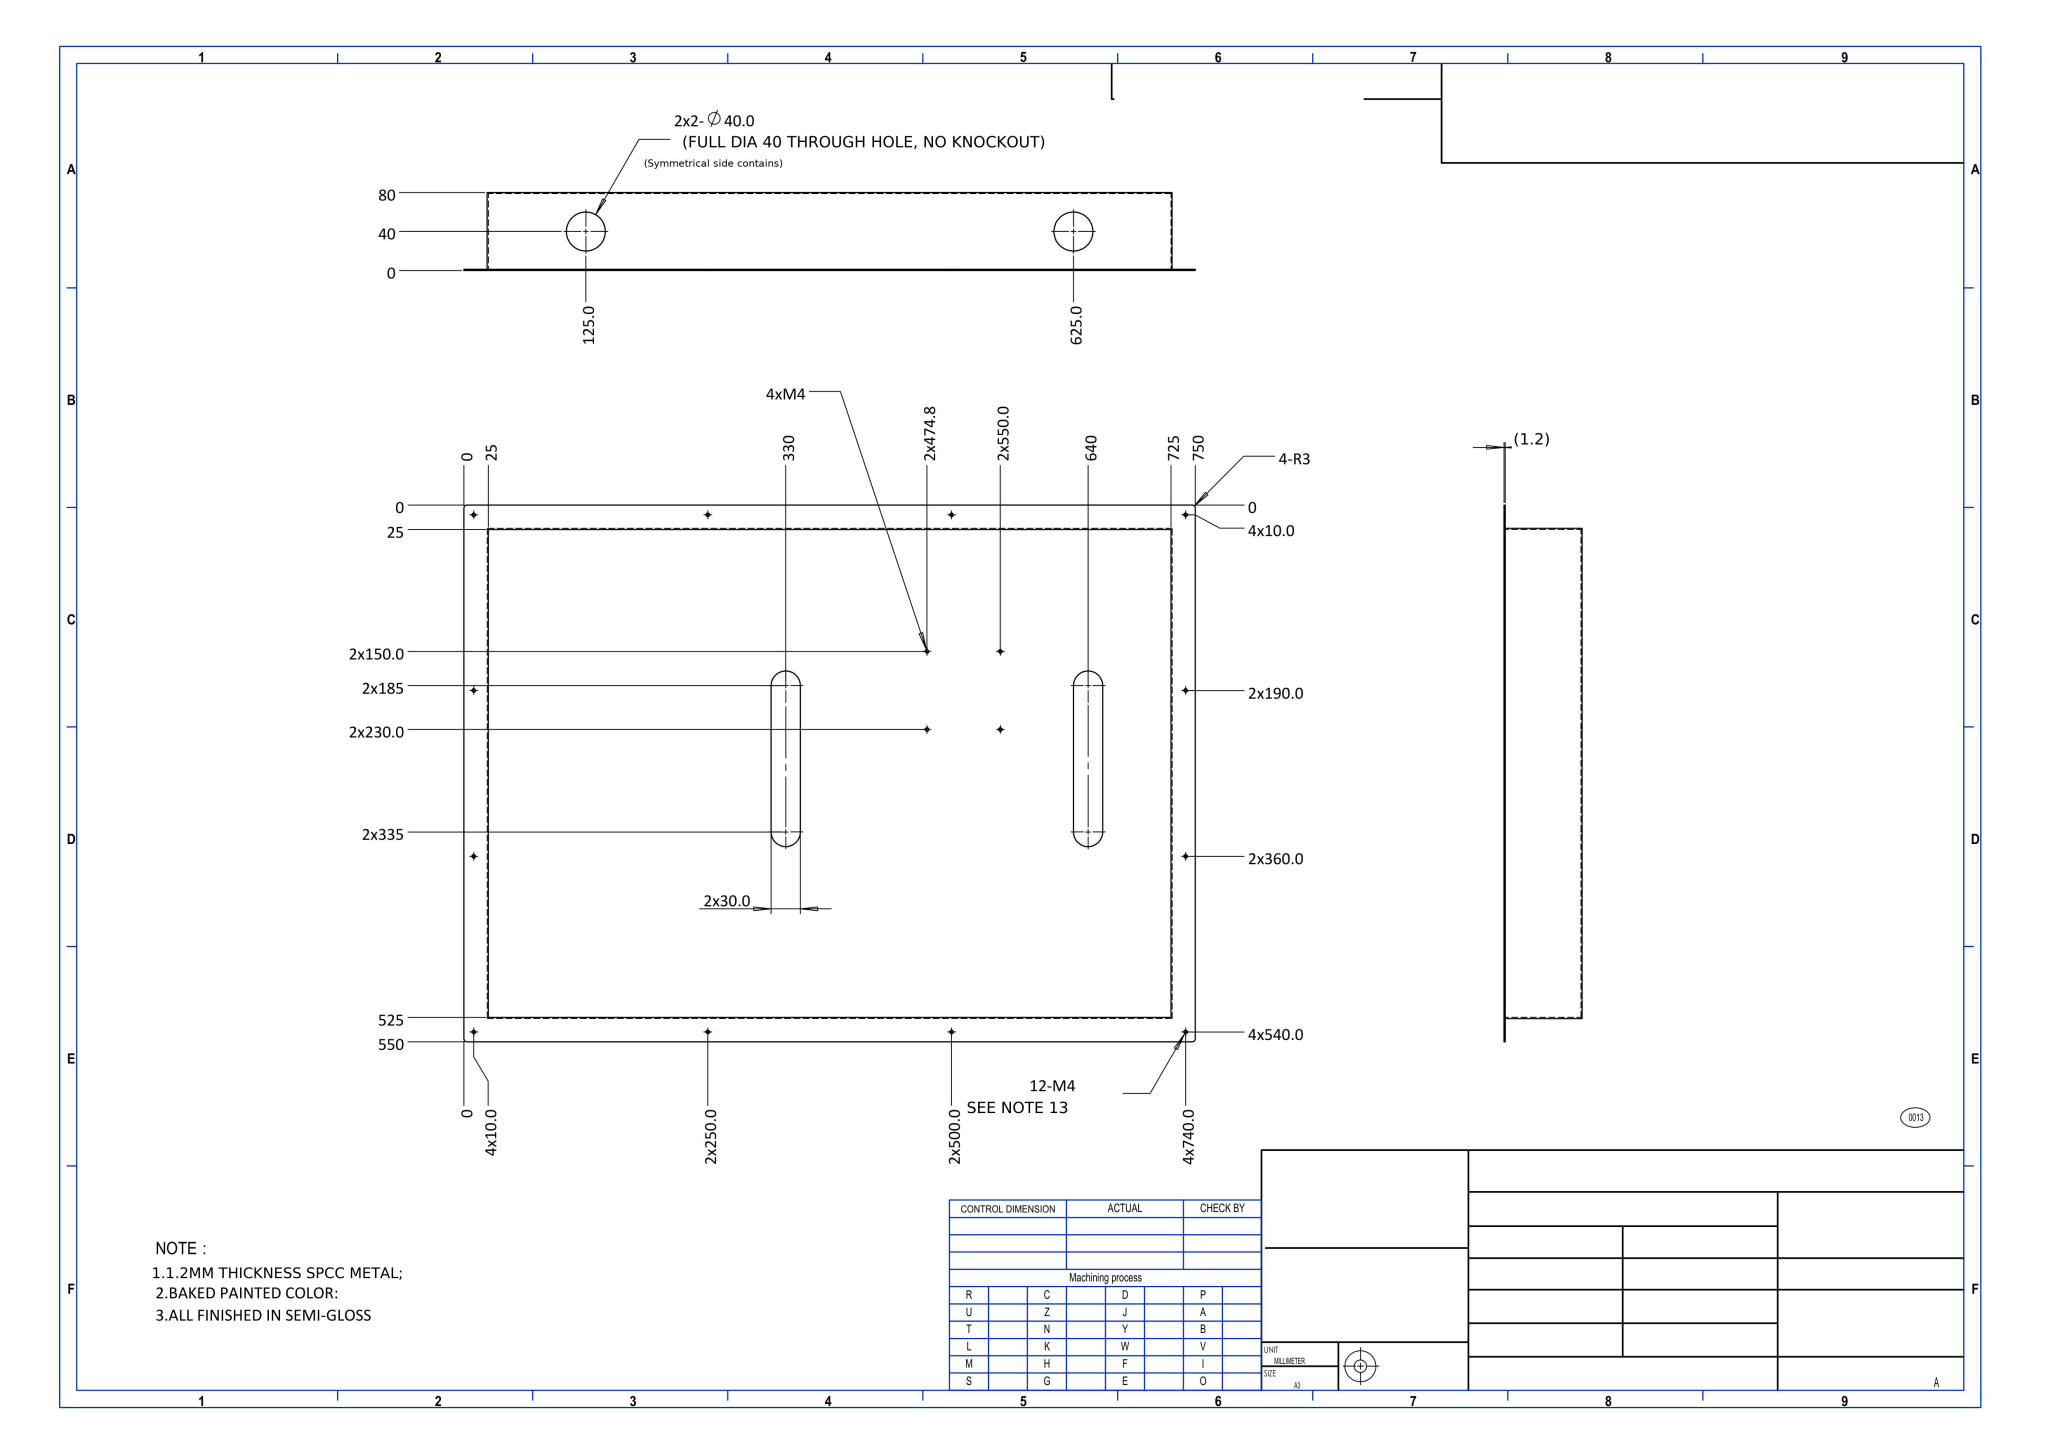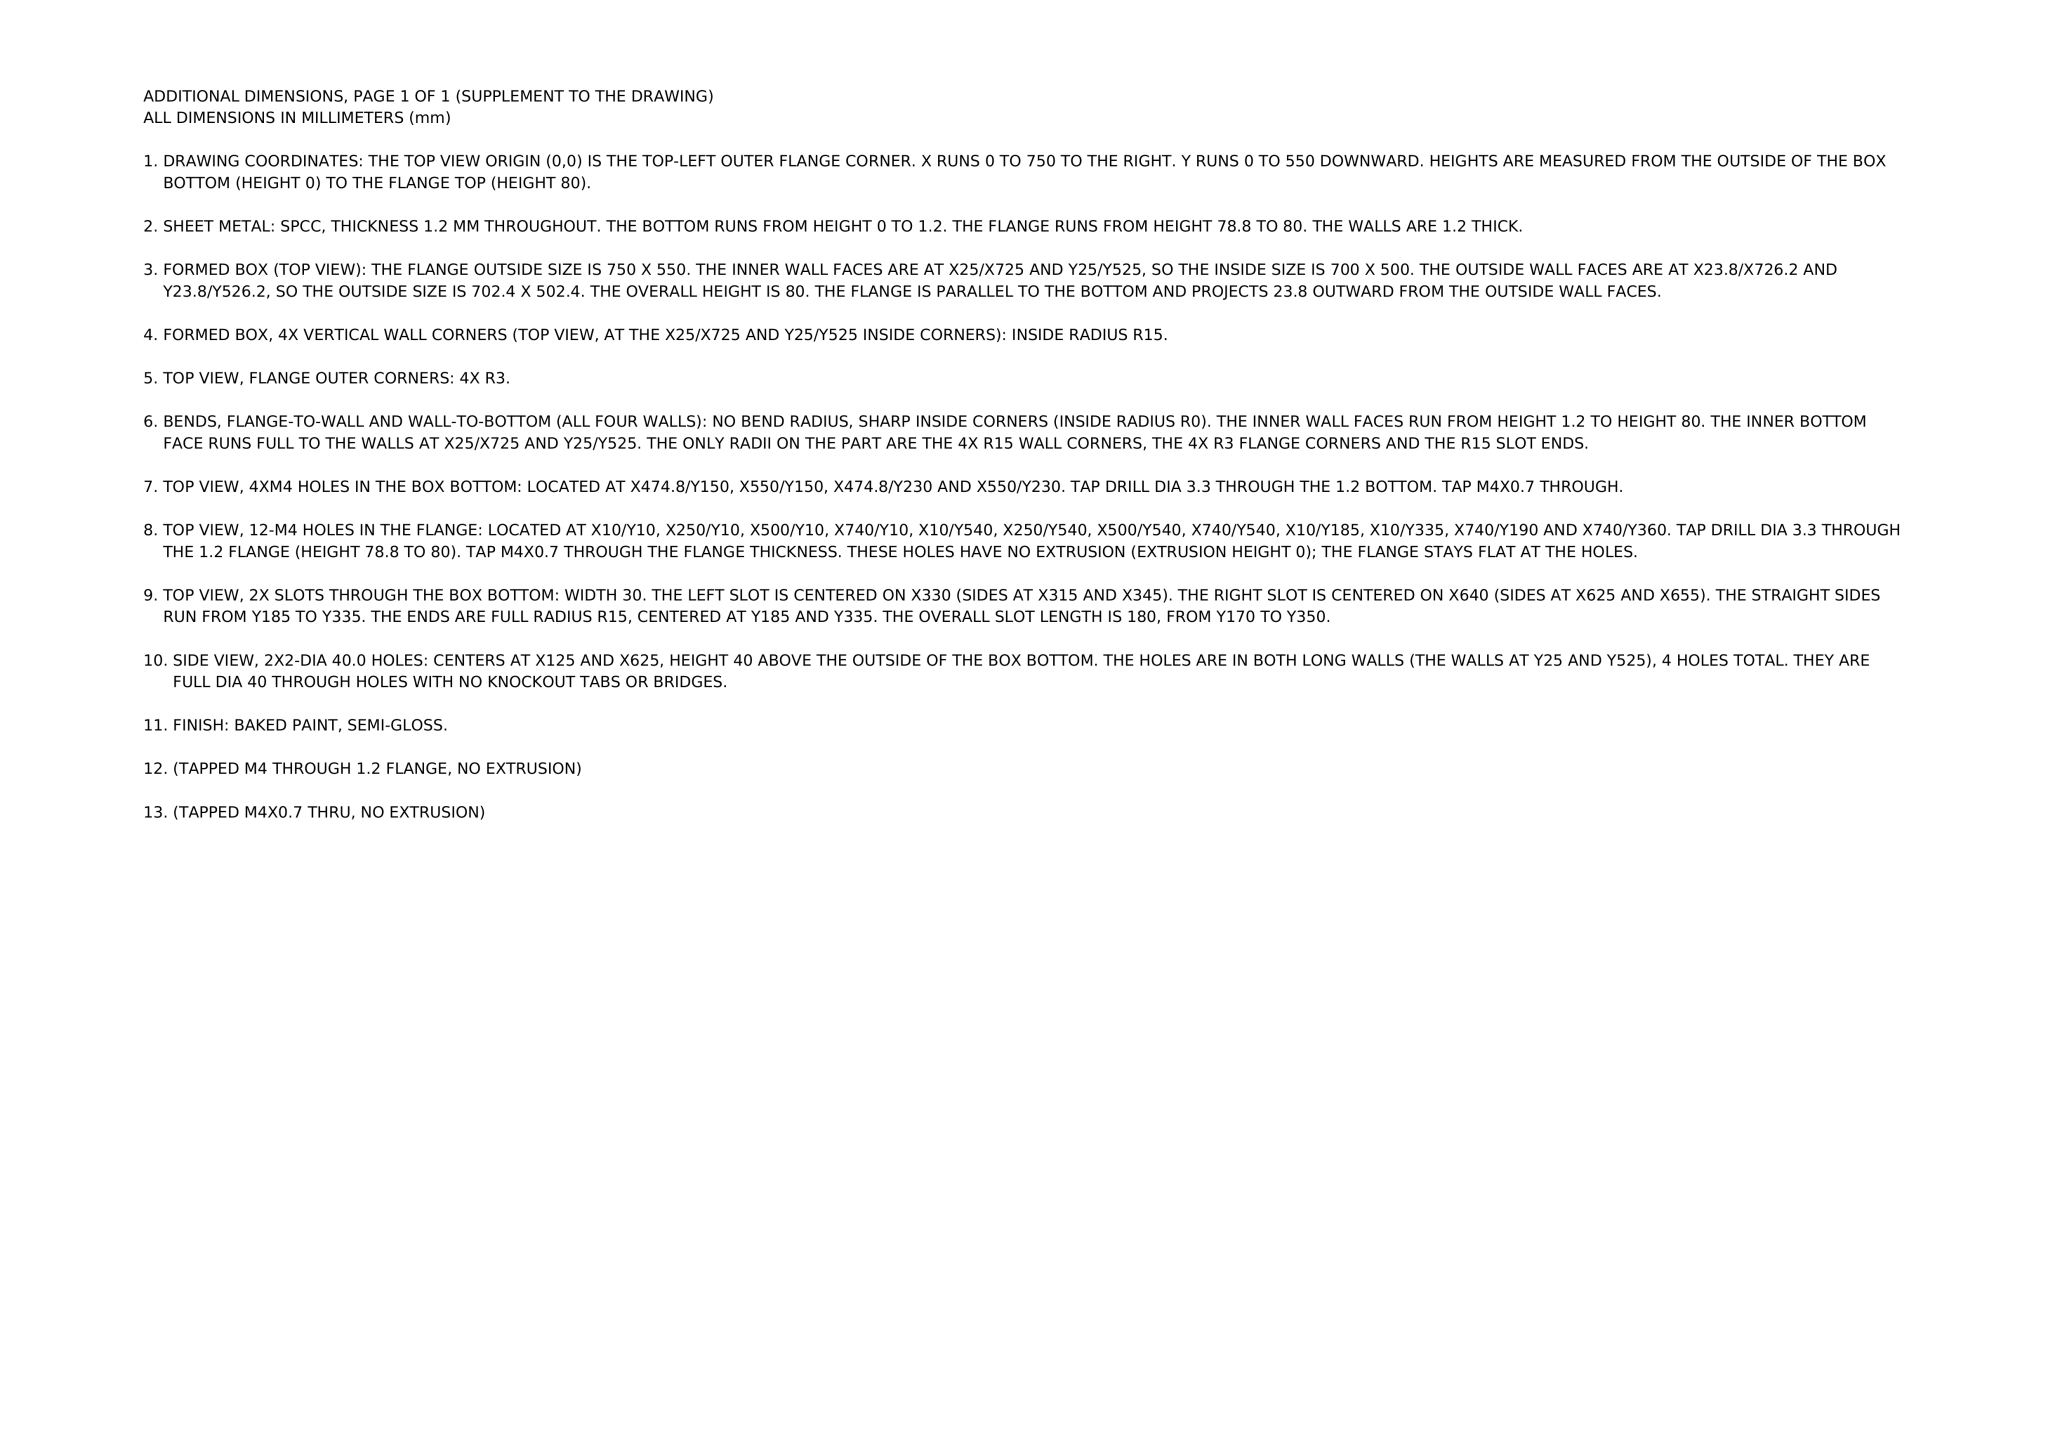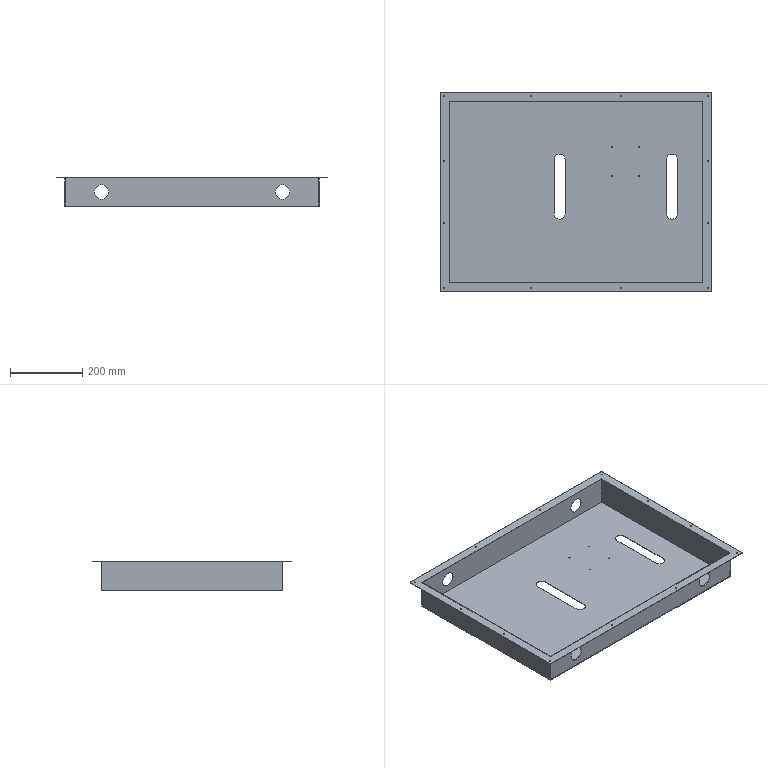Part | NX | mm | 1 solid | 68 faces | box 750 x 550 x 80 mm | volume 703696 mm3 | cylinder 48 | plane 20 | commonest cylinder face diameters 3.3 x32 40 x8 6 x4 30 x4